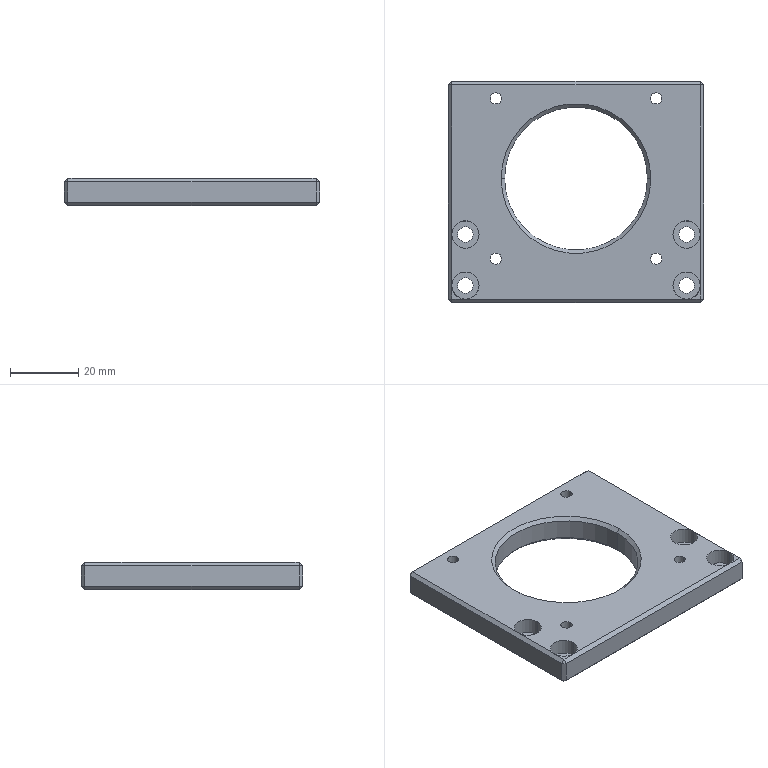Component | SolidWorks | SL010-RightStreamline-1-1_SL010-BeltMotorAssembly-1-1_SL010-LXFB-0102007-1-1 | 1 solid | 62 faces | box 75 x 65 x 8 mm | volume 26077 mm3 | plane 32 | cylinder 26 | cone 4 | commonest cylinder face diameters 8 x8 4.5 x8 3.3 x8 42 x2 | material Aluminum-6061
build123d program:
from build123d import *

# Parameters (mm, degrees)
SKETCH1_W                                          = 75
SKETCH1_H                                          = 65
BOSS_EXTRUDE1_DEPTH                                = 8
M4_TAPPED_HOLE1_D                                  = 3.3
SKETCH4_R                                          = 21
CUT_EXTRUDE1_DEPTH                                 = 8
CHAMFER1_SIZE                                      = 1
HOLE_SIZE_ACCORDING_TO_TYPE_OF_HEXAGON_D           = 4.5
HOLE_SIZE_ACCORDING_TO_TYPE_OF_HEXAGON_CBORE_D     = 8
HOLE_SIZE_ACCORDING_TO_TYPE_OF_HEXAGON_CBORE_DEPTH = 4.6


with BuildPart() as part:
    # Sketch1 → Boss-Extrude1 (new body)
    with BuildSketch(Plane.XY):
        Rectangle(SKETCH1_W, SKETCH1_H)
    extrude(amount=BOSS_EXTRUDE1_DEPTH)

    # M4 Tapped Hole1 (through all)
    with Locations(Plane.XY.offset(8)):
        with Locations((-23.55, 27.5), (-23.55, -19.6), (23.55, -19.6), (23.55, 27.5)):
            Hole(M4_TAPPED_HOLE1_D / 2)

    # Sketch4 → Cut-Extrude1 (cut)
    with BuildSketch(Plane.XY.offset(8)):
        with Locations((0, 3.95)):
            Circle(SKETCH4_R)
    extrude(amount=-CUT_EXTRUDE1_DEPTH, mode=Mode.SUBTRACT)

    # Chamfer1
    chamfer1_edges = [part.edges().sort_by_distance(p)[0] for p in [
        (37.5, 0, 8),
        (0, 32.5, 8),
        (-21, 3.95, 0),
        (-21, 3.95, 8),
        (-37.5, 0, 8),
        (0, 32.5, 0),
        (37.5, 0, 0),
        (0, -32.5, 0),
        (-37.5, 0, 0),
        (0, -32.5, 8),
        (-37.5, 32.5, 4),
        (37.5, 32.5, 4),
        (37.5, -32.5, 4),
        (-37.5, -32.5, 4),
    ]]
    chamfer(chamfer1_edges, length=CHAMFER1_SIZE)

    # Hole Size_ according to_Type of Hexagon (through all)
    with Locations(Plane.XY.offset(8)):
        with Locations((-32.5, -12.5), (-32.5, -27.5)):
            hole_size_according_to_type_of_hexagon = CounterBoreHole(HOLE_SIZE_ACCORDING_TO_TYPE_OF_HEXAGON_D / 2, HOLE_SIZE_ACCORDING_TO_TYPE_OF_HEXAGON_CBORE_D / 2, HOLE_SIZE_ACCORDING_TO_TYPE_OF_HEXAGON_CBORE_DEPTH)

    # Mirror1: Hole Size_ according to_Type of Hexagon across plane
    add(hole_size_according_to_type_of_hexagon.mirror(Plane(origin=(0, 0, 0), x_dir=(0, 0, 1), z_dir=(1, 0, 0))), mode=Mode.SUBTRACT)


solid = part.part

# Placed as in the assembly
solid = solid.moved(Location((-580, -195.404, -296.035), (0, 0, 0)))